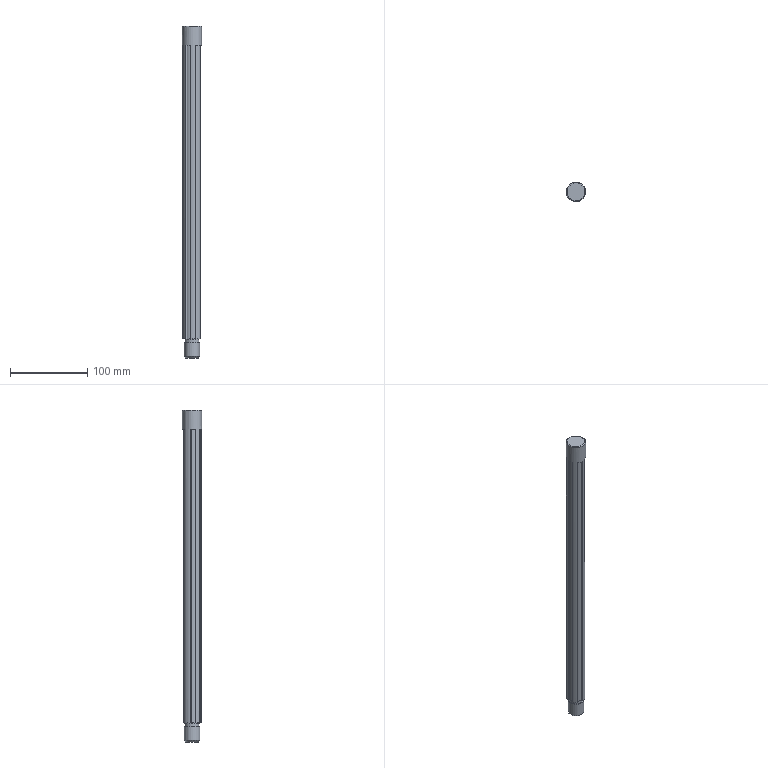Component | NX | CA6140-ZHOU12-HUAJIANZHOU | 1 solid | 22 faces | volume 174532 mm3 | plane 13 | cylinder 6 | torus 2 | cone 1 | commonest cylinder face diameters 22 x3 20 x1 18 x1 25 x1